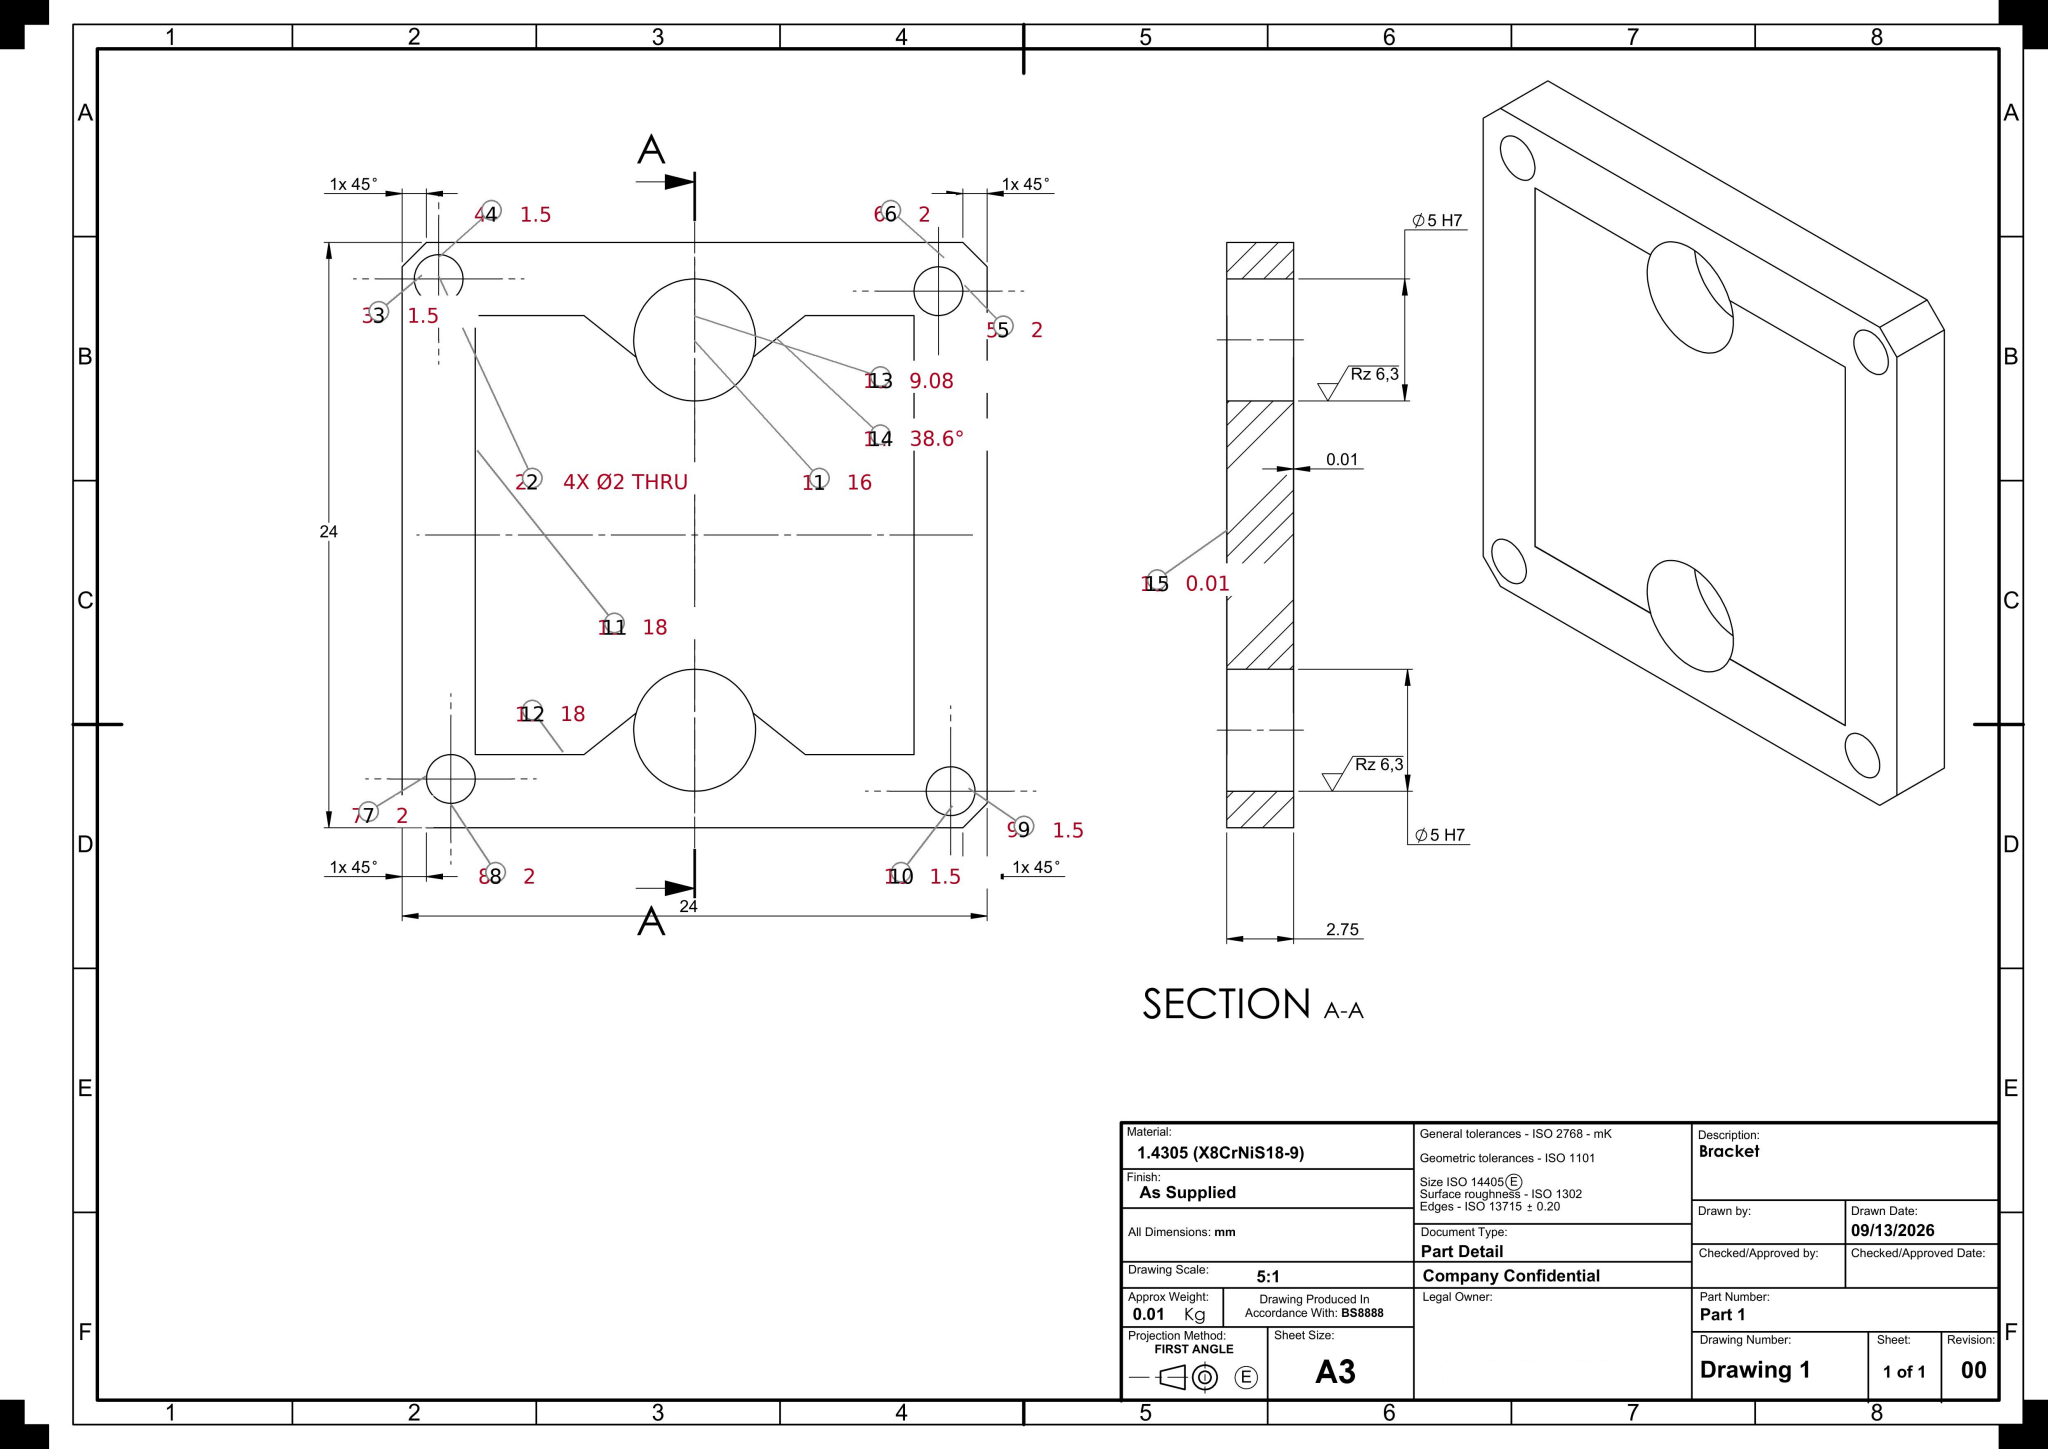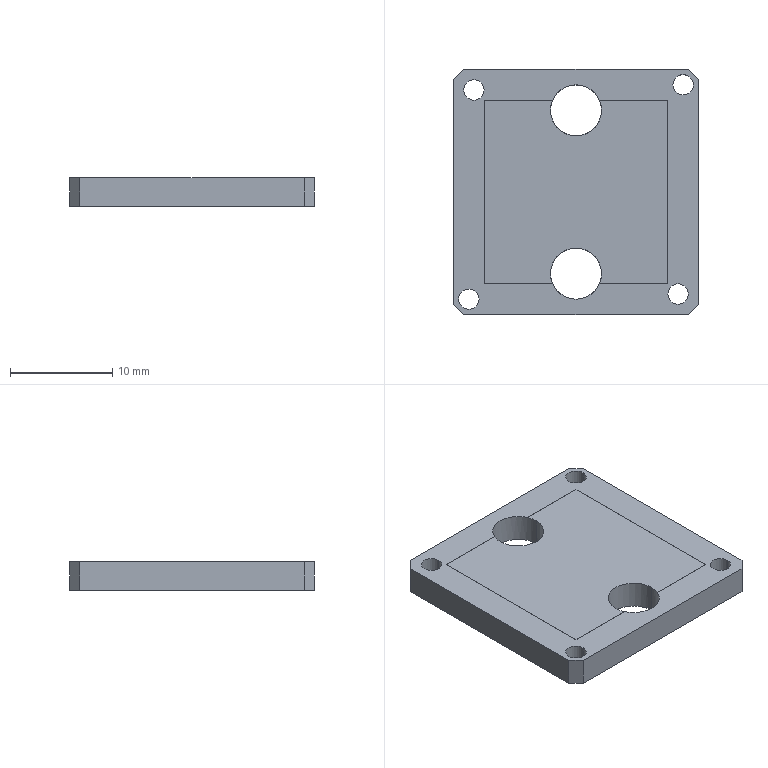Part | SolidWorks | mm | 1 solid | 40 faces | box 24 x 24 x 2.75 mm | volume 1430 mm3 | plane 28 | cylinder 12 | commonest cylinder face diameters 2 x8 5 x4